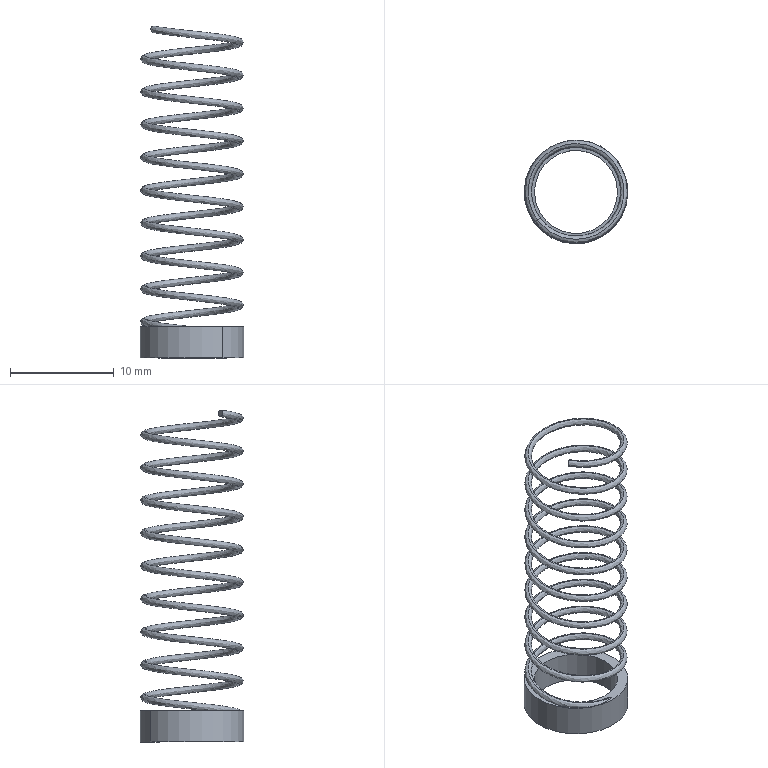Component | SolidWorks | YWY-D10-L35-1 | 1 solid | 9 faces | volume 172 mm3 | cylinder 4 | plane 3 | spline 2 | commonest cylinder face diameters 8 x2 10 x2